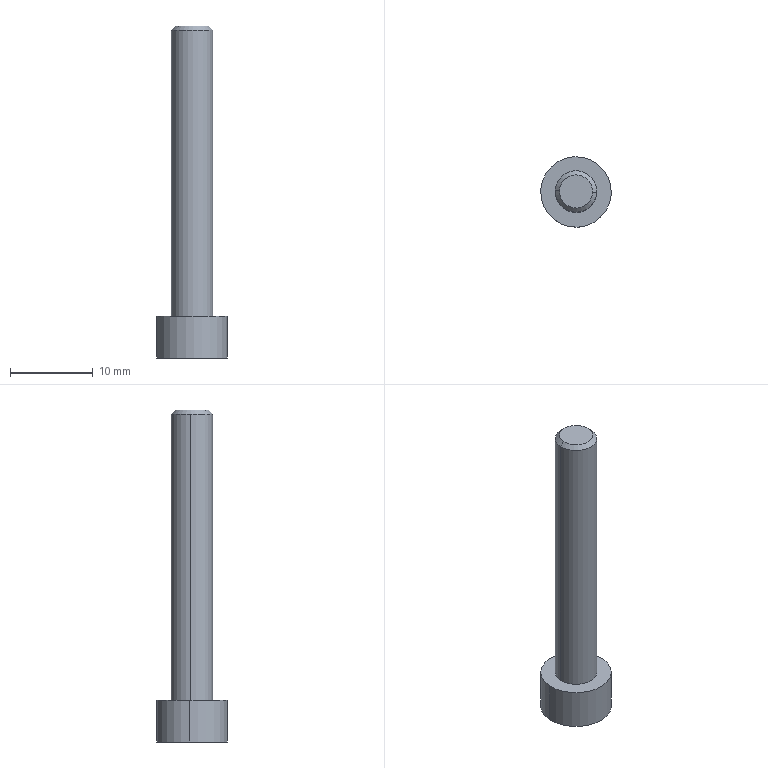Component | SolidWorks | ScrewM5X35-1 | 1 solid | 9 faces | box 8.5 x 8.5 x 40 mm | volume 969 mm3 | cylinder 4 | plane 3 | cone 2 | commonest cylinder face diameters 5 x2 8.5 x2
build123d program:
from build123d import *

# Parameters (mm, degrees)
CHAMFER1_SIZE = 0.5


with BuildPart() as part:
    # Sketch1 → Revolve1 (revolve)
    with BuildSketch(Plane.XY, mode=Mode.PRIVATE) as revolve1_sk:
        Polygon((0, 0), (-4.25, 0), (-4.25, -5), (-2.5, -5), (-2.5, -40), (0, -40), align=None)
    revolve(revolve1_sk.sketch.rotate(Axis((0, 56.699, 0), (0, -1, 0)), 270), axis=Axis((0, 56.699, 0), (0, -1, 0)))

    # Chamfer1
    chamfer1_edges = [part.edges().sort_by_distance(p)[0] for p in [
        (0, -40, -2.5),
    ]]
    chamfer(chamfer1_edges, length=CHAMFER1_SIZE)


solid = part.part

# Placed as in the assembly
solid = solid.moved(Location((23.266, 33.799, 22), (-90, 0, 0)))
STEP:
#1=CARTESIAN_POINT('',(0.8374,1.336,2.441));
#2=VERTEX_POINT('',#1);
#3=CARTESIAN_POINT('',(0.9946,1.326,2.441));
#4=VERTEX_POINT('',#3);
#5=CARTESIAN_POINT('',(0.916,1.331,2.441));
#6=DIRECTION('',(0.,-0.,1.));
#7=DIRECTION('',(-0.9981,0.06151,0.));
#8=AXIS2_PLACEMENT_3D('',#5,#6,#7);
#9=CIRCLE('',#8,0.07874);
#10=EDGE_CURVE('',#2,#4,#9,.T.);
#11=ORIENTED_EDGE('',*,*,#10,.F.);
#12=CARTESIAN_POINT('',(0.8178,1.337,2.421));
#13=VERTEX_POINT('',#12);
#14=CARTESIAN_POINT('',(0.8178,1.337,2.421));
#15=DIRECTION('',(-0.7058,0.04349,-0.7071));
#16=VECTOR('',#15,39.37);
#17=LINE('',#14,#16);
#18=EDGE_CURVE('',#2,#13,#17,.T.);
#19=ORIENTED_EDGE('',*,*,#18,.T.);
#20=CARTESIAN_POINT('',(1.014,1.325,2.421));
#21=VERTEX_POINT('',#20);
#22=CARTESIAN_POINT('',(0.916,1.331,2.421));
#23=DIRECTION('',(-0.,0.,-1.));
#24=DIRECTION('',(-0.9981,0.06151,0.));
#25=AXIS2_PLACEMENT_3D('',#22,#23,#24);
#26=CIRCLE('',#25,0.09843);
#27=EDGE_CURVE('',#21,#13,#26,.T.);
#28=ORIENTED_EDGE('',*,*,#27,.F.);
#29=CARTESIAN_POINT('',(1.014,1.325,2.421));
#30=DIRECTION('',(0.7058,-0.04349,-0.7071));
#31=VECTOR('',#30,39.37);
#32=LINE('',#29,#31);
#33=EDGE_CURVE('',#4,#21,#32,.T.);
#34=ORIENTED_EDGE('',*,*,#33,.F.);
#35=EDGE_LOOP('',(#11,#19,#28,#34));
#36=FACE_OUTER_BOUND('',#35,.T.);
#37=CARTESIAN_POINT('',(0.916,1.331,2.421));
#38=DIRECTION('',(-0.,0.,-1.));
#39=DIRECTION('',(0.9981,-0.06151,0.));
#40=AXIS2_PLACEMENT_3D('',#37,#38,#39);
#41=CONICAL_SURFACE('',#40,0.09843,0.7854);
#42=ADVANCED_FACE('',(#36),#41,.T.);
#43=ORIENTED_EDGE('',*,*,#27,.T.);
#44=CARTESIAN_POINT('',(0.8178,1.337,1.063));
#45=VERTEX_POINT('',#44);
#46=CARTESIAN_POINT('',(0.8178,1.337,-1.366));
#47=DIRECTION('',(-0.,0.,-1.));
#48=VECTOR('',#47,39.37);
#49=LINE('',#46,#48);
#50=EDGE_CURVE('',#13,#45,#49,.T.);
#51=ORIENTED_EDGE('',*,*,#50,.T.);
#52=CARTESIAN_POINT('',(1.014,1.325,1.063));
#53=VERTEX_POINT('',#52);
#54=CARTESIAN_POINT('',(0.916,1.331,1.063));
#55=DIRECTION('',(-0.,0.,-1.));
#56=DIRECTION('',(0.9981,-0.06151,0.));
#57=AXIS2_PLACEMENT_3D('',#54,#55,#56);
#58=CIRCLE('',#57,0.09843);
#59=EDGE_CURVE('',#53,#45,#58,.T.);
#60=ORIENTED_EDGE('',*,*,#59,.F.);
#61=CARTESIAN_POINT('',(1.014,1.325,-1.366));
#62=DIRECTION('',(-0.,0.,-1.));
#63=VECTOR('',#62,39.37);
#64=LINE('',#61,#63);
#65=EDGE_CURVE('',#21,#53,#64,.T.);
#66=ORIENTED_EDGE('',*,*,#65,.F.);
#67=EDGE_LOOP('',(#43,#51,#60,#66));
#68=FACE_OUTER_BOUND('',#67,.T.);
#69=CARTESIAN_POINT('',(0.916,1.331,-1.366));
#70=DIRECTION('',(-0.,0.,-1.));
#71=DIRECTION('',(0.9981,-0.06151,0.));
#72=AXIS2_PLACEMENT_3D('',#69,#70,#71);
#73=CYLINDRICAL_SURFACE('',#72,0.09843);
#74=ADVANCED_FACE('',(#68),#73,.T.);
#75=CARTESIAN_POINT('',(1.083,1.32,1.063));
#76=VERTEX_POINT('',#75);
#77=CARTESIAN_POINT('',(0.749,1.341,1.063));
#78=VERTEX_POINT('',#77);
#79=CARTESIAN_POINT('',(0.916,1.331,1.063));
#80=DIRECTION('',(-0.,0.,-1.));
#81=DIRECTION('',(0.9981,-0.06151,0.));
#82=AXIS2_PLACEMENT_3D('',#79,#80,#81);
#83=CIRCLE('',#82,0.1673);
#84=EDGE_CURVE('',#76,#78,#83,.T.);
#85=ORIENTED_EDGE('',*,*,#84,.T.);
#86=CARTESIAN_POINT('',(0.749,1.341,0.8661));
#87=VERTEX_POINT('',#86);
#88=CARTESIAN_POINT('',(0.749,1.341,-1.366));
#89=DIRECTION('',(-0.,0.,-1.));
#90=VECTOR('',#89,39.37);
#91=LINE('',#88,#90);
#92=EDGE_CURVE('',#78,#87,#91,.T.);
#93=ORIENTED_EDGE('',*,*,#92,.T.);
#94=CARTESIAN_POINT('',(1.083,1.32,0.8661));
#95=VERTEX_POINT('',#94);
#96=CARTESIAN_POINT('',(0.916,1.331,0.8661));
#97=DIRECTION('',(-0.,0.,-1.));
#98=DIRECTION('',(0.9981,-0.06151,0.));
#99=AXIS2_PLACEMENT_3D('',#96,#97,#98);
#100=CIRCLE('',#99,0.1673);
#101=EDGE_CURVE('',#95,#87,#100,.T.);
#102=ORIENTED_EDGE('',*,*,#101,.F.);
#103=CARTESIAN_POINT('',(1.083,1.32,-1.366));
#104=DIRECTION('',(-0.,0.,-1.));
#105=VECTOR('',#104,39.37);
#106=LINE('',#103,#105);
#107=EDGE_CURVE('',#76,#95,#106,.T.);
#108=ORIENTED_EDGE('',*,*,#107,.F.);
#109=EDGE_LOOP('',(#85,#93,#102,#108));
#110=FACE_OUTER_BOUND('',#109,.T.);
#111=CARTESIAN_POINT('',(0.916,1.331,-1.366));
#112=DIRECTION('',(-0.,0.,-1.));
#113=DIRECTION('',(0.9981,-0.06151,0.));
#114=AXIS2_PLACEMENT_3D('',#111,#112,#113);
#115=CYLINDRICAL_SURFACE('',#114,0.1673);
#116=ADVANCED_FACE('',(#110),#115,.T.);
#117=ORIENTED_EDGE('',*,*,#101,.T.);
#118=CARTESIAN_POINT('',(0.916,1.331,0.8661));
#119=DIRECTION('',(-0.,0.,-1.));
#120=DIRECTION('',(0.9981,-0.06151,0.));
#121=AXIS2_PLACEMENT_3D('',#118,#119,#120);
#122=CIRCLE('',#121,0.1673);
#123=EDGE_CURVE('',#87,#95,#122,.T.);
#124=ORIENTED_EDGE('',*,*,#123,.T.);
#125=EDGE_LOOP('',(#117,#124));
#126=FACE_OUTER_BOUND('',#125,.T.);
#127=CARTESIAN_POINT('',(0.916,1.331,0.8661));
#128=DIRECTION('',(0.,0.,-1.));
#129=DIRECTION('',(0.9981,-0.06151,0.));
#130=AXIS2_PLACEMENT_3D('',#127,#128,#129);
#131=PLANE('',#130);
#132=ADVANCED_FACE('',(#126),#131,.T.);
#133=ORIENTED_EDGE('',*,*,#92,.F.);
#134=CARTESIAN_POINT('',(0.916,1.331,1.063));
#135=DIRECTION('',(-0.,0.,-1.));
#136=DIRECTION('',(0.9981,-0.06151,0.));
#137=AXIS2_PLACEMENT_3D('',#134,#135,#136);
#138=CIRCLE('',#137,0.1673);
#139=EDGE_CURVE('',#78,#76,#138,.T.);
#140=ORIENTED_EDGE('',*,*,#139,.T.);
#141=ORIENTED_EDGE('',*,*,#107,.T.);
#142=ORIENTED_EDGE('',*,*,#123,.F.);
#143=EDGE_LOOP('',(#133,#140,#141,#142));
#144=FACE_OUTER_BOUND('',#143,.T.);
#145=CARTESIAN_POINT('',(0.916,1.331,-1.366));
#146=DIRECTION('',(-0.,0.,-1.));
#147=DIRECTION('',(0.9981,-0.06151,0.));
#148=AXIS2_PLACEMENT_3D('',#145,#146,#147);
#149=CYLINDRICAL_SURFACE('',#148,0.1673);
#150=ADVANCED_FACE('',(#144),#149,.T.);
#151=ORIENTED_EDGE('',*,*,#59,.T.);
#152=CARTESIAN_POINT('',(0.916,1.331,1.063));
#153=DIRECTION('',(-0.,0.,-1.));
#154=DIRECTION('',(0.9981,-0.06151,0.));
#155=AXIS2_PLACEMENT_3D('',#152,#153,#154);
#156=CIRCLE('',#155,0.09843);
#157=EDGE_CURVE('',#45,#53,#156,.T.);
#158=ORIENTED_EDGE('',*,*,#157,.T.);
#159=EDGE_LOOP('',(#151,#158));
#160=FACE_BOUND('',#159,.T.);
#161=ORIENTED_EDGE('',*,*,#84,.F.);
#162=ORIENTED_EDGE('',*,*,#139,.F.);
#163=EDGE_LOOP('',(#161,#162));
#164=FACE_OUTER_BOUND('',#163,.T.);
#165=CARTESIAN_POINT('',(0.9263,1.498,1.063));
#166=DIRECTION('',(-0.,-0.,1.));
#167=DIRECTION('',(-0.9981,0.06151,-0.));
#168=AXIS2_PLACEMENT_3D('',#165,#166,#167);
#169=PLANE('',#168);
#170=ADVANCED_FACE('',(#160,#164),#169,.T.);
#171=ORIENTED_EDGE('',*,*,#50,.F.);
#172=CARTESIAN_POINT('',(0.916,1.331,2.421));
#173=DIRECTION('',(-0.,0.,-1.));
#174=DIRECTION('',(-0.9981,0.06151,0.));
#175=AXIS2_PLACEMENT_3D('',#172,#173,#174);
#176=CIRCLE('',#175,0.09843);
#177=EDGE_CURVE('',#13,#21,#176,.T.);
#178=ORIENTED_EDGE('',*,*,#177,.T.);
#179=ORIENTED_EDGE('',*,*,#65,.T.);
#180=ORIENTED_EDGE('',*,*,#157,.F.);
#181=EDGE_LOOP('',(#171,#178,#179,#180));
#182=FACE_OUTER_BOUND('',#181,.T.);
#183=CARTESIAN_POINT('',(0.916,1.331,-1.366));
#184=DIRECTION('',(-0.,0.,-1.));
#185=DIRECTION('',(0.9981,-0.06151,0.));
#186=AXIS2_PLACEMENT_3D('',#183,#184,#185);
#187=CYLINDRICAL_SURFACE('',#186,0.09843);
#188=ADVANCED_FACE('',(#182),#187,.T.);
#189=CARTESIAN_POINT('',(0.916,1.331,2.441));
#190=DIRECTION('',(0.,-0.,1.));
#191=DIRECTION('',(-0.9981,0.06151,0.));
#192=AXIS2_PLACEMENT_3D('',#189,#190,#191);
#193=CIRCLE('',#192,0.07874);
#194=EDGE_CURVE('',#4,#2,#193,.T.);
#195=ORIENTED_EDGE('',*,*,#194,.T.);
#196=ORIENTED_EDGE('',*,*,#10,.T.);
#197=EDGE_LOOP('',(#195,#196));
#198=FACE_OUTER_BOUND('',#197,.T.);
#199=CARTESIAN_POINT('',(0.922,1.429,2.441));
#200=DIRECTION('',(-0.,-0.,1.));
#201=DIRECTION('',(-0.9981,0.06151,-0.));
#202=AXIS2_PLACEMENT_3D('',#199,#200,#201);
#203=PLANE('',#202);
#204=ADVANCED_FACE('',(#198),#203,.T.);
#205=ORIENTED_EDGE('',*,*,#18,.F.);
#206=ORIENTED_EDGE('',*,*,#194,.F.);
#207=ORIENTED_EDGE('',*,*,#33,.T.);
#208=ORIENTED_EDGE('',*,*,#177,.F.);
#209=EDGE_LOOP('',(#205,#206,#207,#208));
#210=FACE_OUTER_BOUND('',#209,.T.);
#211=CARTESIAN_POINT('',(0.916,1.331,2.421));
#212=DIRECTION('',(-0.,0.,-1.));
#213=DIRECTION('',(0.9981,-0.06151,0.));
#214=AXIS2_PLACEMENT_3D('',#211,#212,#213);
#215=CONICAL_SURFACE('',#214,0.09843,0.7854);
#216=ADVANCED_FACE('',(#210),#215,.T.);
#217=CLOSED_SHELL('',(#42,#74,#116,#132,#150,#170,#188,#204,#216));
#218=MANIFOLD_SOLID_BREP('',#217);
#219=CARTESIAN_POINT('',(0.,0.,0.));
#220=DIRECTION('',(0.,0.,1.));
#221=DIRECTION('',(1.,0.,0.));
#222=AXIS2_PLACEMENT_3D('',#219,#220,#221);
#223=(LENGTH_UNIT()NAMED_UNIT(*)SI_UNIT($,.METRE.));
#224=LENGTH_MEASURE_WITH_UNIT(LENGTH_MEASURE(0.0254),#223);
#225=DIMENSIONAL_EXPONENTS(1.,0.,0.,0.,0.,0.,0.);
#226=(CONVERSION_BASED_UNIT('',#224)LENGTH_UNIT()NAMED_UNIT(#225));
#227=UNCERTAINTY_MEASURE_WITH_UNIT(LENGTH_MEASURE(0.00001),#226,'','');
#228=(NAMED_UNIT(*)PLANE_ANGLE_UNIT()SI_UNIT($,.RADIAN.));
#229=(NAMED_UNIT(*)SI_UNIT($,.STERADIAN.)SOLID_ANGLE_UNIT());
#230=(GEOMETRIC_REPRESENTATION_CONTEXT(3)GLOBAL_UNCERTAINTY_ASSIGNED_CONTEXT((#227))GLOBAL_UNIT_ASSIGNED_CONTEXT((#226,#228,#229))REPRESENTATION_CONTEXT('',''));
#231=ADVANCED_BREP_SHAPE_REPRESENTATION('',(#218,#222),#230);
#232=COLOUR_RGB('',0.7922,0.8196,0.9333);
#233=FILL_AREA_STYLE_COLOUR('',#232);
#234=FILL_AREA_STYLE('',(#233));
#235=SURFACE_STYLE_FILL_AREA(#234);
#236=SURFACE_SIDE_STYLE('',(#235));
#237=SURFACE_STYLE_USAGE(.BOTH.,#236);
#238=PRESENTATION_STYLE_ASSIGNMENT((#237));
#239=STYLED_ITEM('',(#238),#218);
#240=PRESENTATION_LAYER_ASSIGNMENT('','',(#239));
#241=(LENGTH_UNIT()NAMED_UNIT(*)SI_UNIT($,.METRE.));
#242=LENGTH_MEASURE_WITH_UNIT(LENGTH_MEASURE(0.0254),#241);
#243=DIMENSIONAL_EXPONENTS(1.,0.,0.,0.,0.,0.,0.);
#244=(CONVERSION_BASED_UNIT('',#242)LENGTH_UNIT()NAMED_UNIT(#243));
#245=UNCERTAINTY_MEASURE_WITH_UNIT(LENGTH_MEASURE(0.00001),#244,'','');
#246=(NAMED_UNIT(*)PLANE_ANGLE_UNIT()SI_UNIT($,.RADIAN.));
#247=(NAMED_UNIT(*)SI_UNIT($,.STERADIAN.)SOLID_ANGLE_UNIT());
#248=(GEOMETRIC_REPRESENTATION_CONTEXT(3)GLOBAL_UNCERTAINTY_ASSIGNED_CONTEXT((#245))GLOBAL_UNIT_ASSIGNED_CONTEXT((#244,#246,#247))REPRESENTATION_CONTEXT('',''));
#249=MECHANICAL_DESIGN_GEOMETRIC_PRESENTATION_REPRESENTATION('',(#239),#248);